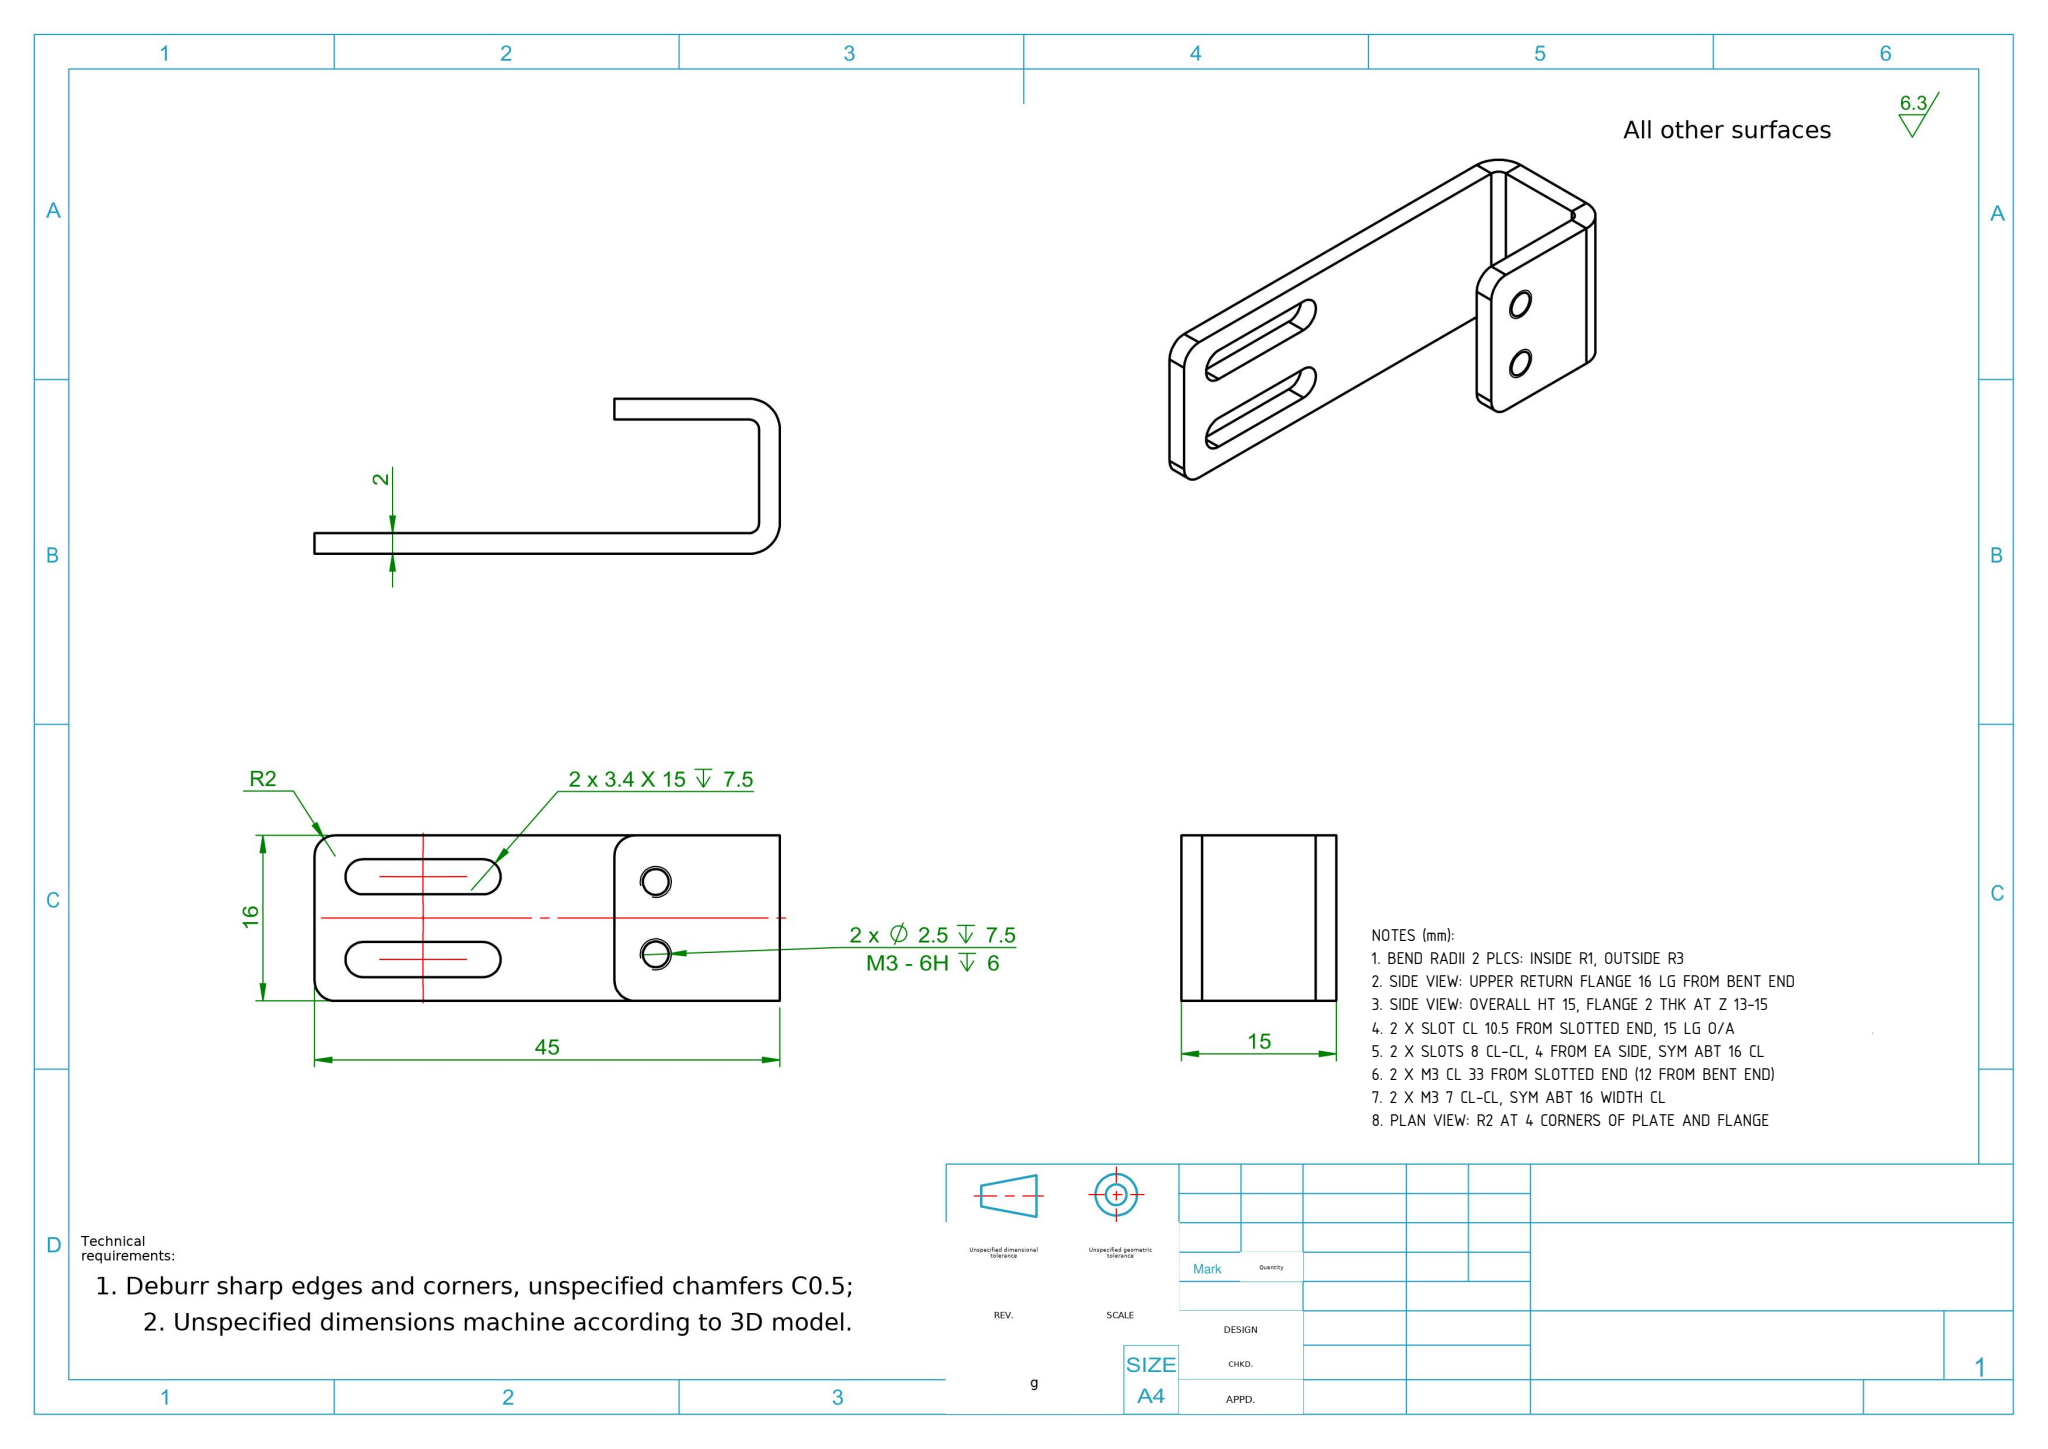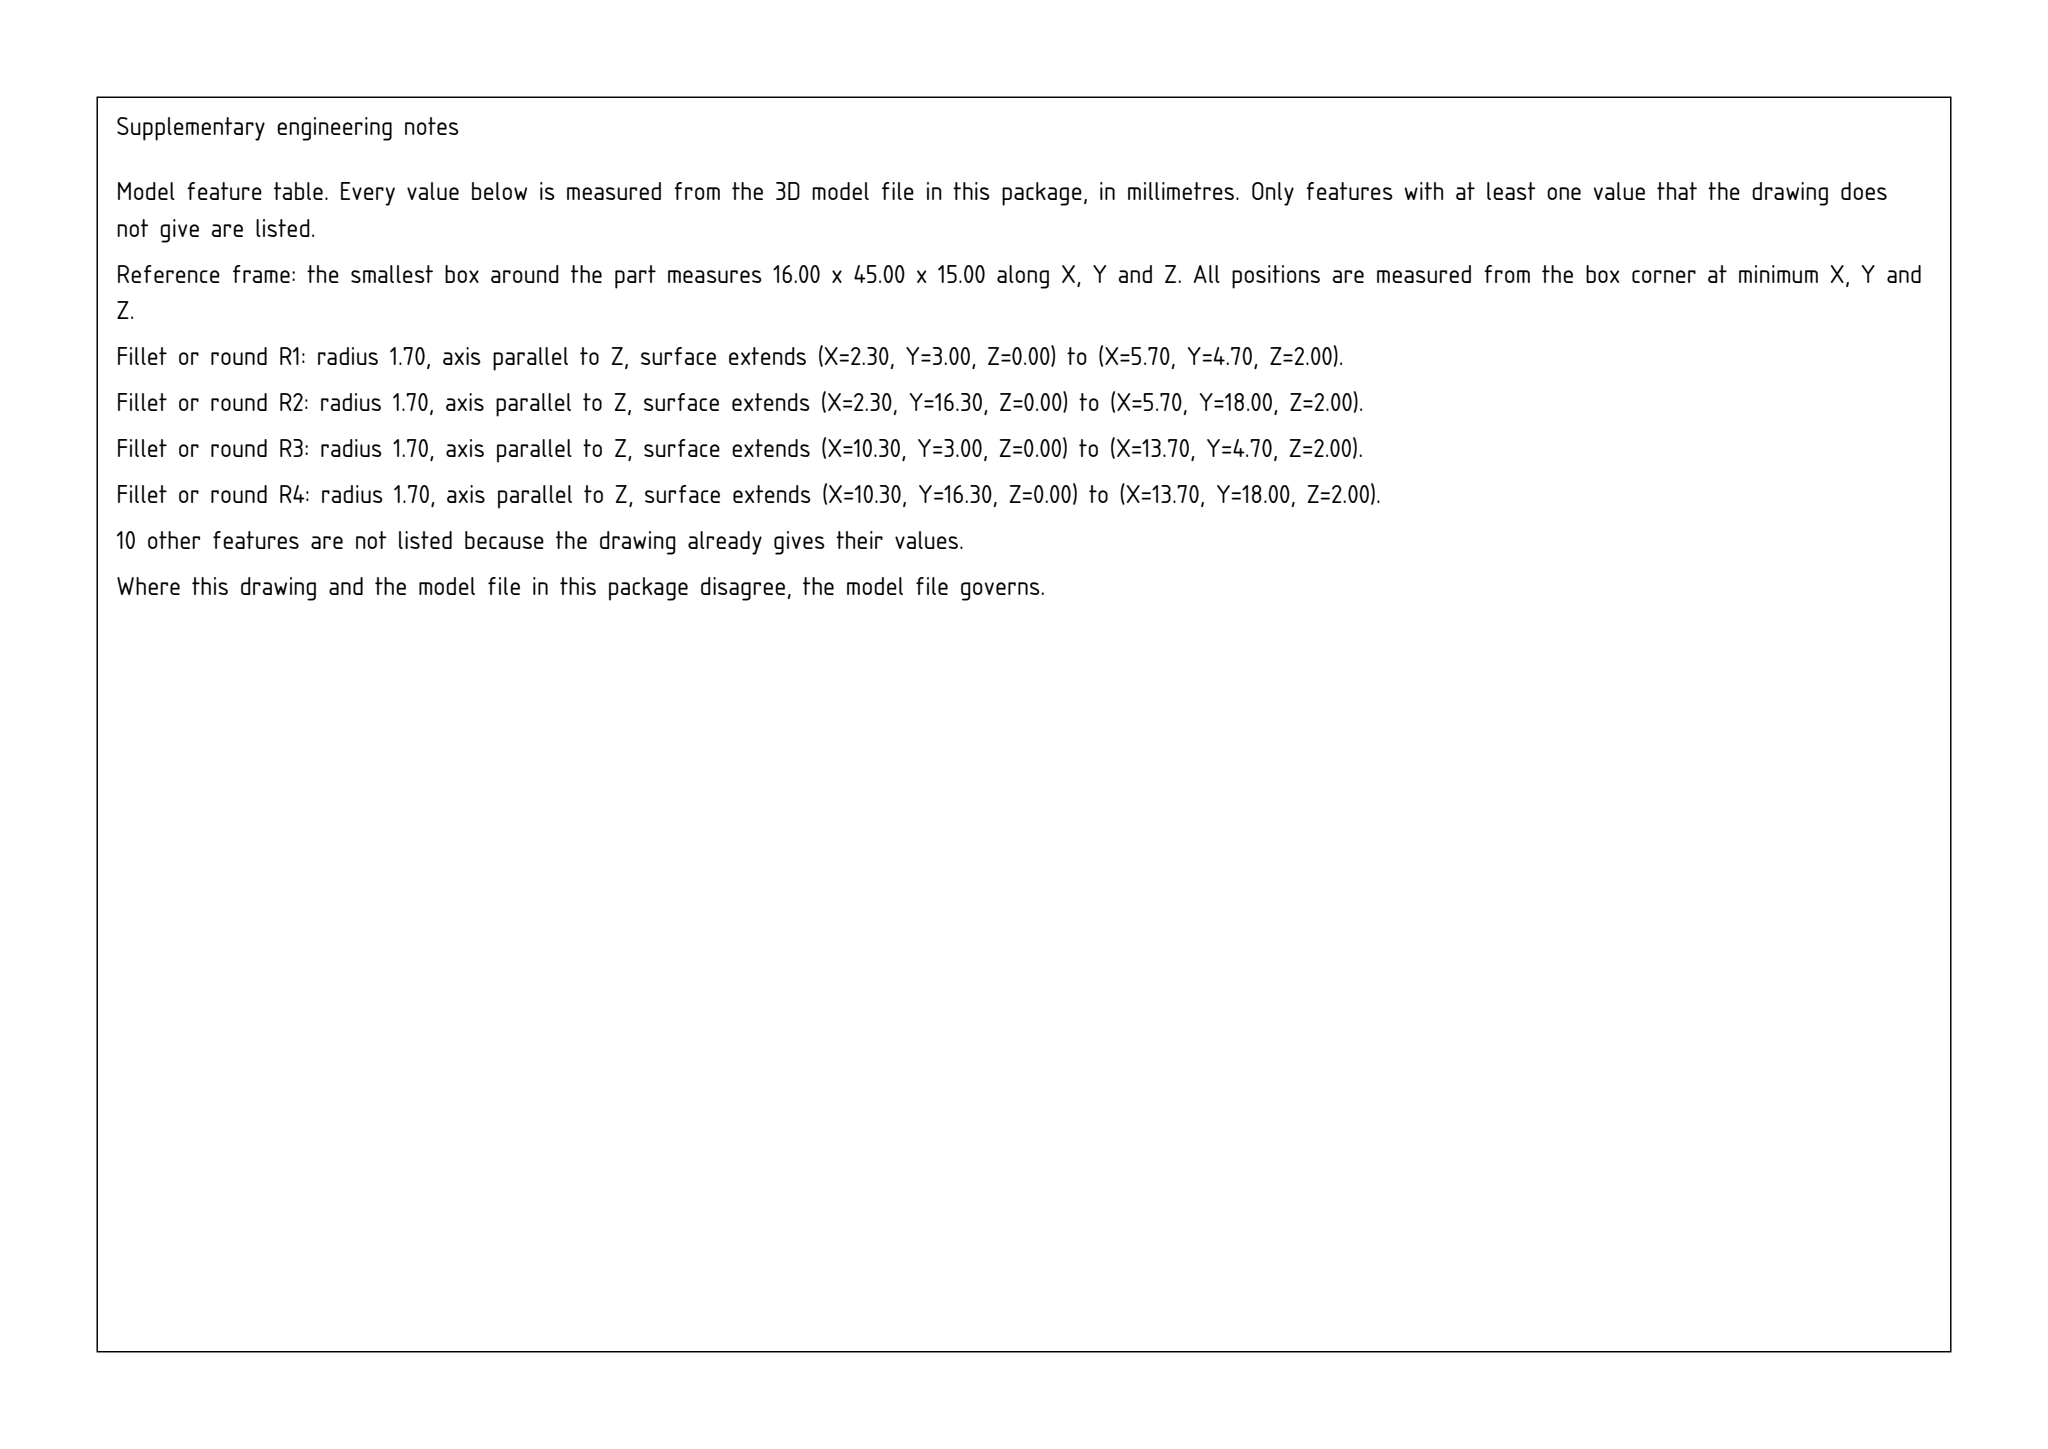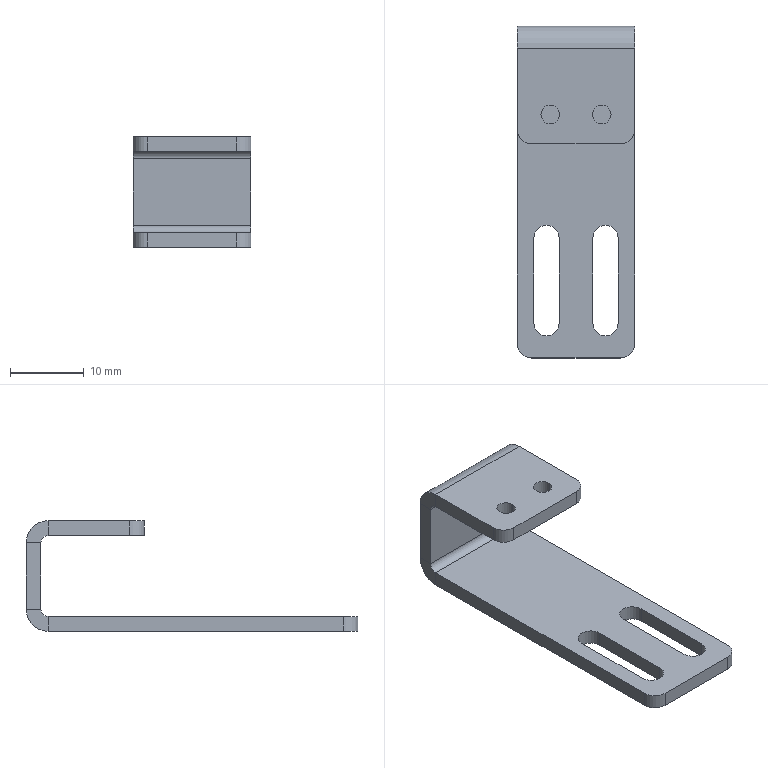Part | SolidWorks | mm | 1 solid | 38 faces | box 16 x 45 x 15 mm | volume 2028 mm3 | plane 22 | cylinder 16 | commonest cylinder face diameters 2.5 x4 3.4 x4 4 x4 6 x2 2 x2
Drawing notes:
BEND RADII 2 PLCS: INSIDE R1, OUTSIDE R3 | from the solid: x-axis cyl dia2 (inner) & dia6 (outer) at y=42,z=3 and y=42,z=12 -> R1 inside / R3 outside
SIDE VIEW: UPPER RETURN FLANGE 16 LG FROM BENT END | from the solid: y-planes 29 and 45; flange free end y=29, bent end y=45 -> 45-29=16
SIDE VIEW: OVERALL HT 15, FLANGE 2 THK AT Z 13-15 | from the solid: bbox z=15; z-planes 0,2,13,15
2 X SLOT CL 10.5 FROM SLOTTED END, 15 LG O/A | from the solid: 3.4 dia ends at y=4.7 & 16.3 -> CL y=10.5, overall 4.7-1.7 to 16.3+1.7 = 15
2 X SLOTS 8 CL-CL, 4 FROM EA SIDE, SYM ABT 16 CL | from the solid: 3.4 slot axes at x=4.0 and x=12.0, bbox x=16
2 X M3 CL 33 FROM SLOTTED END (12 FROM BENT END) | from the solid: 2.5 dia z-axis holes at y=33; bent end y=45
2 X M3 7 CL-CL, SYM ABT 16 WIDTH CL | from the solid: 2.5 dia holes at x=4.5 and x=11.5 -> 7 apart, mean x=8
PLAN VIEW: R2 AT 4 CORNERS OF PLATE AND FLANGE | from the solid: 4.0 dia z-axis cyls at (2,2),(14,2),(2,31),(14,31) -> R2